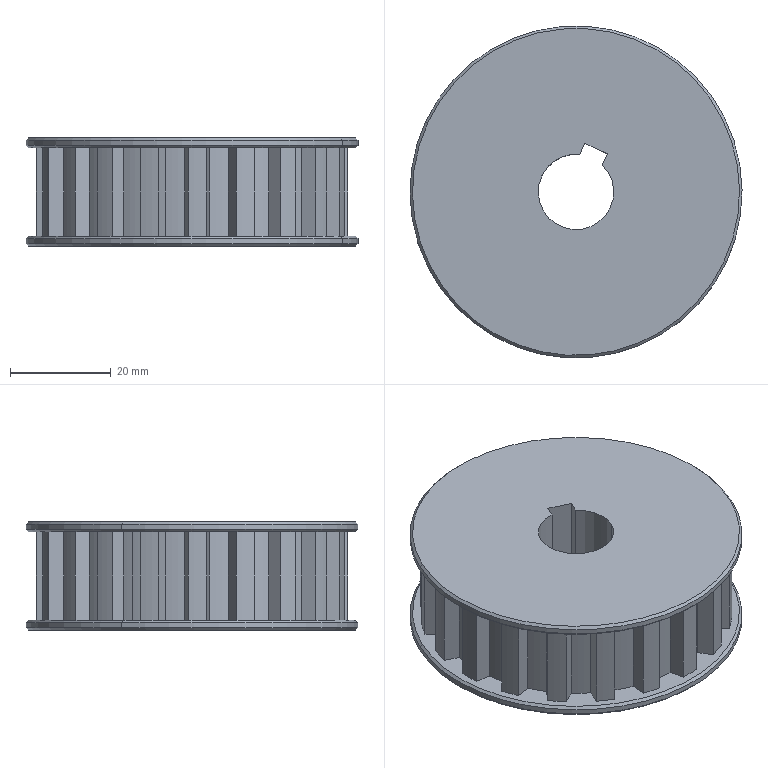Component | SolidWorks | DoubleFilmTransport-1_DriveWheel-1 | 1 solid | 103 faces | volume 57195 mm3 | cylinder 48 | plane 47 | cone 8 | commonest cylinder face diameters 56 x21 62 x20 66 x4 15 x3